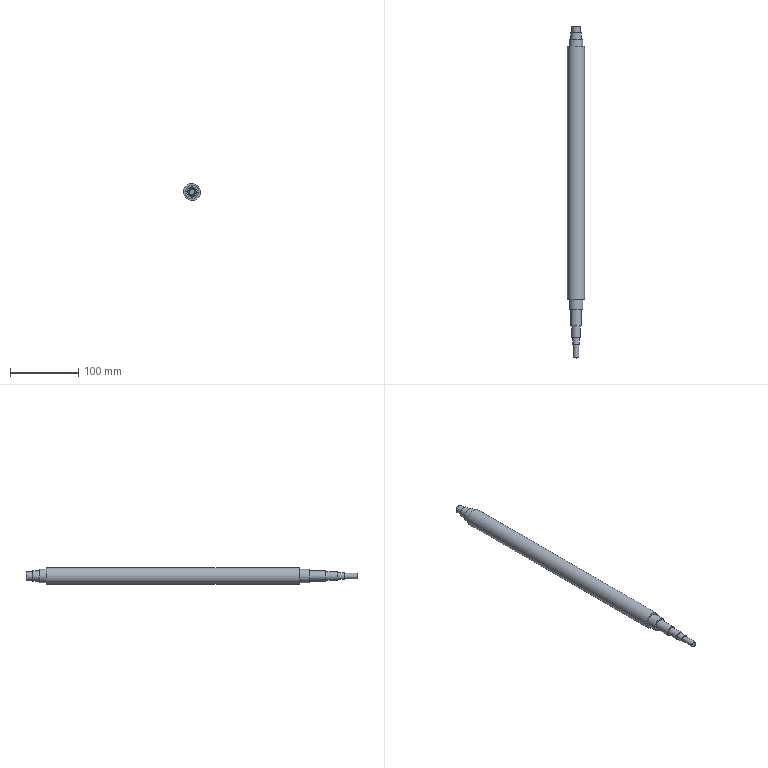Component | NX | Y_LEADSCREW | 1 solid | 19 faces | box 25 x 486 x 25 mm | volume 200330 mm3 | plane 10 | cylinder 9 | commonest cylinder face diameters 12 x2 15 x2 20 x2 8 x1 10 x1 25 x1
STEP:
#1=CARTESIAN_POINT('',(0.,0.,0.));
#2=DIRECTION('',(0.,0.,1.));
#3=DIRECTION('',(1.,0.,0.));
#4=AXIS2_PLACEMENT_3D('',#1,#2,#3);
#5=CARTESIAN_POINT('',(626.907,146.698,-1470.977));
#6=VERTEX_POINT('',#5);
#7=CARTESIAN_POINT('',(630.189,146.698,-1476.));
#8=DIRECTION('',(0.,-1.,0.));
#9=DIRECTION('',(-0.5469,0.,0.8372));
#10=AXIS2_PLACEMENT_3D('',#7,#8,#9);
#11=CIRCLE('',#10,6.);
#12=CARTESIAN_POINT('',(630.189,146.698,-1476.));
#13=DIRECTION('',(0.,-1.,0.));
#14=DIRECTION('',(-0.5469,0.,0.8372));
#15=AXIS2_PLACEMENT_3D('',#12,#13,#14);
#16=PLANE('',#15);
#17=CARTESIAN_POINT('',(0.,0.));
#18=DIRECTION('',(1.,0.));
#19=AXIS2_PLACEMENT_2D('',#17,#18);
#20=CIRCLE('',#19,6.);
#21=(GEOMETRIC_REPRESENTATION_CONTEXT(2)PARAMETRIC_REPRESENTATION_CONTEXT()REPRESENTATION_CONTEXT('',''));
#22=DEFINITIONAL_REPRESENTATION('',(#20),#21);
#23=PCURVE('',#16,#22);
#24=CARTESIAN_POINT('',(630.189,-68.302,-1476.));
#25=DIRECTION('',(0.,-1.,0.));
#26=DIRECTION('',(-0.5469,0.,0.8372));
#27=AXIS2_PLACEMENT_3D('',#24,#25,#26);
#28=CYLINDRICAL_SURFACE('',#27,6.);
#29=CARTESIAN_POINT('',(0.,-215.));
#30=DIRECTION('',(1.,0.));
#31=VECTOR('',#30,1.);
#32=LINE('',#29,#31);
#33=(GEOMETRIC_REPRESENTATION_CONTEXT(2)PARAMETRIC_REPRESENTATION_CONTEXT()REPRESENTATION_CONTEXT('',''));
#34=DEFINITIONAL_REPRESENTATION('',(#32),#33);
#35=PCURVE('',#28,#34);
#36=SURFACE_CURVE('',#11,(#23,#35),.PCURVE_S1.);
#37=EDGE_CURVE('',#6,#6,#36,.T.);
#38=ORIENTED_EDGE('',*,*,#37,.F.);
#39=EDGE_LOOP('',(#38));
#40=FACE_BOUND('',#39,.T.);
#41=ADVANCED_FACE('',(#40),#16,.F.);
#42=CARTESIAN_POINT('',(628.001,-339.302,-1472.651));
#43=VERTEX_POINT('',#42);
#44=CARTESIAN_POINT('',(630.189,-339.302,-1476.));
#45=DIRECTION('',(0.,-1.,0.));
#46=DIRECTION('',(-0.5469,0.,0.8372));
#47=AXIS2_PLACEMENT_3D('',#44,#45,#46);
#48=CIRCLE('',#47,4.);
#49=CARTESIAN_POINT('',(630.189,-339.302,-1476.));
#50=DIRECTION('',(0.,-1.,0.));
#51=DIRECTION('',(-0.5469,0.,0.8372));
#52=AXIS2_PLACEMENT_3D('',#49,#50,#51);
#53=PLANE('',#52);
#54=CARTESIAN_POINT('',(0.,0.));
#55=DIRECTION('',(1.,-0.));
#56=AXIS2_PLACEMENT_2D('',#54,#55);
#57=CIRCLE('',#56,4.);
#58=(GEOMETRIC_REPRESENTATION_CONTEXT(2)PARAMETRIC_REPRESENTATION_CONTEXT()REPRESENTATION_CONTEXT('',''));
#59=DEFINITIONAL_REPRESENTATION('',(#57),#58);
#60=PCURVE('',#53,#59);
#61=CARTESIAN_POINT('',(630.189,-68.302,-1476.));
#62=DIRECTION('',(0.,-1.,0.));
#63=DIRECTION('',(-0.5469,0.,0.8372));
#64=AXIS2_PLACEMENT_3D('',#61,#62,#63);
#65=CYLINDRICAL_SURFACE('',#64,4.);
#66=CARTESIAN_POINT('',(0.,271.));
#67=DIRECTION('',(1.,0.));
#68=VECTOR('',#67,1.);
#69=LINE('',#66,#68);
#70=(GEOMETRIC_REPRESENTATION_CONTEXT(2)PARAMETRIC_REPRESENTATION_CONTEXT()REPRESENTATION_CONTEXT('',''));
#71=DEFINITIONAL_REPRESENTATION('',(#69),#70);
#72=PCURVE('',#65,#71);
#73=SURFACE_CURVE('',#48,(#60,#72),.PCURVE_S1.);
#74=EDGE_CURVE('',#43,#43,#73,.T.);
#75=ORIENTED_EDGE('',*,*,#74,.T.);
#76=EDGE_LOOP('',(#75));
#77=FACE_BOUND('',#76,.T.);
#78=ADVANCED_FACE('',(#77),#53,.T.);
#79=ORIENTED_EDGE('',*,*,#74,.F.);
#80=CARTESIAN_POINT('',(628.001,-319.302,-1472.651));
#81=VERTEX_POINT('',#80);
#82=CARTESIAN_POINT('',(628.001,-319.302,-1472.651));
#83=CARTESIAN_POINT('',(628.001,-339.302,-1472.651));
#84=B_SPLINE_CURVE_WITH_KNOTS('',1,(#82,#83),.UNSPECIFIED.,.F.,.F.,(2,2),(251.,271.),.PIECEWISE_BEZIER_KNOTS.);
#85=CARTESIAN_POINT('',(0.,0.));
#86=DIRECTION('',(0.,1.));
#87=VECTOR('',#86,1.);
#88=LINE('',#85,#87);
#89=(GEOMETRIC_REPRESENTATION_CONTEXT(2)PARAMETRIC_REPRESENTATION_CONTEXT()REPRESENTATION_CONTEXT('',''));
#90=DEFINITIONAL_REPRESENTATION('',(#88),#89);
#91=PCURVE('',#65,#90);
#92=CARTESIAN_POINT('',(6.283,0.));
#93=DIRECTION('',(0.,1.));
#94=VECTOR('',#93,1.);
#95=LINE('',#92,#94);
#96=(GEOMETRIC_REPRESENTATION_CONTEXT(2)PARAMETRIC_REPRESENTATION_CONTEXT()REPRESENTATION_CONTEXT('',''));
#97=DEFINITIONAL_REPRESENTATION('',(#95),#96);
#98=PCURVE('',#65,#97);
#99=SEAM_CURVE('',#84,(#91,#98),.PCURVE_S1.);
#100=EDGE_CURVE('',#81,#43,#99,.T.);
#101=ORIENTED_EDGE('',*,*,#100,.F.);
#102=CARTESIAN_POINT('',(630.189,-319.302,-1476.));
#103=DIRECTION('',(0.,-1.,0.));
#104=DIRECTION('',(-0.5469,0.,0.8372));
#105=AXIS2_PLACEMENT_3D('',#102,#103,#104);
#106=CIRCLE('',#105,4.);
#107=CARTESIAN_POINT('',(0.,251.));
#108=DIRECTION('',(1.,0.));
#109=VECTOR('',#108,1.);
#110=LINE('',#107,#109);
#111=(GEOMETRIC_REPRESENTATION_CONTEXT(2)PARAMETRIC_REPRESENTATION_CONTEXT()REPRESENTATION_CONTEXT('',''));
#112=DEFINITIONAL_REPRESENTATION('',(#110),#111);
#113=PCURVE('',#65,#112);
#114=CARTESIAN_POINT('',(632.924,-319.302,-1480.186));
#115=DIRECTION('',(0.,1.,0.));
#116=DIRECTION('',(0.5469,0.,-0.8372));
#117=AXIS2_PLACEMENT_3D('',#114,#115,#116);
#118=PLANE('',#117);
#119=CARTESIAN_POINT('',(-9.,-0.));
#120=CARTESIAN_POINT('',(-9.,6.928));
#121=CARTESIAN_POINT('',(-3.,3.464));
#122=CARTESIAN_POINT('',(3.,-0.));
#123=CARTESIAN_POINT('',(-3.,-3.464));
#124=CARTESIAN_POINT('',(-9.,-6.928));
#125=CARTESIAN_POINT('',(-9.,-0.));
#126=(BOUNDED_CURVE()B_SPLINE_CURVE(2,(#119,#120,#121,#122,#123,#124,#125),.UNSPECIFIED.,.T.,.F.)B_SPLINE_CURVE_WITH_KNOTS((1,2,2,2,2,1),(-2.094,0.,2.094,4.189,6.283,8.378),.UNSPECIFIED.)CURVE()GEOMETRIC_REPRESENTATION_ITEM()RATIONAL_B_SPLINE_CURVE((1.,0.5,1.,0.5,1.,0.5,1.))REPRESENTATION_ITEM(''));
#127=(GEOMETRIC_REPRESENTATION_CONTEXT(2)PARAMETRIC_REPRESENTATION_CONTEXT()REPRESENTATION_CONTEXT('',''));
#128=DEFINITIONAL_REPRESENTATION('',(#126),#127);
#129=PCURVE('',#118,#128);
#130=SURFACE_CURVE('',#106,(#113,#129),.PCURVE_S1.);
#131=EDGE_CURVE('',#81,#81,#130,.T.);
#132=ORIENTED_EDGE('',*,*,#131,.T.);
#133=ORIENTED_EDGE('',*,*,#100,.T.);
#134=EDGE_LOOP('',(#79,#101,#132,#133));
#135=FACE_BOUND('',#134,.T.);
#136=ADVANCED_FACE('',(#135),#65,.T.);
#137=ORIENTED_EDGE('',*,*,#131,.F.);
#138=EDGE_LOOP('',(#137));
#139=FACE_BOUND('',#138,.T.);
#140=CARTESIAN_POINT('',(627.454,-319.302,-1471.814));
#141=VERTEX_POINT('',#140);
#142=CARTESIAN_POINT('',(630.189,-319.302,-1476.));
#143=DIRECTION('',(0.,-1.,0.));
#144=DIRECTION('',(-0.5469,0.,0.8372));
#145=AXIS2_PLACEMENT_3D('',#142,#143,#144);
#146=CIRCLE('',#145,5.);
#147=CARTESIAN_POINT('',(-10.,-0.));
#148=CARTESIAN_POINT('',(-10.,8.66));
#149=CARTESIAN_POINT('',(-2.5,4.33));
#150=CARTESIAN_POINT('',(5.,-0.));
#151=CARTESIAN_POINT('',(-2.5,-4.33));
#152=CARTESIAN_POINT('',(-10.,-8.66));
#153=CARTESIAN_POINT('',(-10.,-0.));
#154=(BOUNDED_CURVE()B_SPLINE_CURVE(2,(#147,#148,#149,#150,#151,#152,#153),.UNSPECIFIED.,.T.,.F.)B_SPLINE_CURVE_WITH_KNOTS((1,2,2,2,2,1),(-2.094,0.,2.094,4.189,6.283,8.378),.UNSPECIFIED.)CURVE()GEOMETRIC_REPRESENTATION_ITEM()RATIONAL_B_SPLINE_CURVE((1.,0.5,1.,0.5,1.,0.5,1.))REPRESENTATION_ITEM(''));
#155=(GEOMETRIC_REPRESENTATION_CONTEXT(2)PARAMETRIC_REPRESENTATION_CONTEXT()REPRESENTATION_CONTEXT('',''));
#156=DEFINITIONAL_REPRESENTATION('',(#154),#155);
#157=PCURVE('',#118,#156);
#158=CARTESIAN_POINT('',(630.189,-68.302,-1476.));
#159=DIRECTION('',(0.,-1.,0.));
#160=DIRECTION('',(-0.5469,0.,0.8372));
#161=AXIS2_PLACEMENT_3D('',#158,#159,#160);
#162=CYLINDRICAL_SURFACE('',#161,5.);
#163=CARTESIAN_POINT('',(0.,251.));
#164=DIRECTION('',(1.,0.));
#165=VECTOR('',#164,1.);
#166=LINE('',#163,#165);
#167=(GEOMETRIC_REPRESENTATION_CONTEXT(2)PARAMETRIC_REPRESENTATION_CONTEXT()REPRESENTATION_CONTEXT('',''));
#168=DEFINITIONAL_REPRESENTATION('',(#166),#167);
#169=PCURVE('',#162,#168);
#170=SURFACE_CURVE('',#146,(#157,#169),.PCURVE_S1.);
#171=EDGE_CURVE('',#141,#141,#170,.T.);
#172=ORIENTED_EDGE('',*,*,#171,.T.);
#173=EDGE_LOOP('',(#172));
#174=FACE_BOUND('',#173,.T.);
#175=ADVANCED_FACE('',(#139,#174),#118,.F.);
#176=ORIENTED_EDGE('',*,*,#171,.F.);
#177=CARTESIAN_POINT('',(627.454,-309.302,-1471.814));
#178=VERTEX_POINT('',#177);
#179=CARTESIAN_POINT('',(627.454,-309.302,-1471.814));
#180=CARTESIAN_POINT('',(627.454,-319.302,-1471.814));
#181=B_SPLINE_CURVE_WITH_KNOTS('',1,(#179,#180),.UNSPECIFIED.,.F.,.F.,(2,2),(241.,251.),.PIECEWISE_BEZIER_KNOTS.);
#182=CARTESIAN_POINT('',(0.,0.));
#183=DIRECTION('',(0.,1.));
#184=VECTOR('',#183,1.);
#185=LINE('',#182,#184);
#186=(GEOMETRIC_REPRESENTATION_CONTEXT(2)PARAMETRIC_REPRESENTATION_CONTEXT()REPRESENTATION_CONTEXT('',''));
#187=DEFINITIONAL_REPRESENTATION('',(#185),#186);
#188=PCURVE('',#162,#187);
#189=CARTESIAN_POINT('',(6.283,0.));
#190=DIRECTION('',(0.,1.));
#191=VECTOR('',#190,1.);
#192=LINE('',#189,#191);
#193=(GEOMETRIC_REPRESENTATION_CONTEXT(2)PARAMETRIC_REPRESENTATION_CONTEXT()REPRESENTATION_CONTEXT('',''));
#194=DEFINITIONAL_REPRESENTATION('',(#192),#193);
#195=PCURVE('',#162,#194);
#196=SEAM_CURVE('',#181,(#188,#195),.PCURVE_S1.);
#197=EDGE_CURVE('',#178,#141,#196,.T.);
#198=ORIENTED_EDGE('',*,*,#197,.F.);
#199=CARTESIAN_POINT('',(630.189,-309.302,-1476.));
#200=DIRECTION('',(0.,-1.,0.));
#201=DIRECTION('',(-0.5469,0.,0.8372));
#202=AXIS2_PLACEMENT_3D('',#199,#200,#201);
#203=CIRCLE('',#202,5.);
#204=CARTESIAN_POINT('',(0.,241.));
#205=DIRECTION('',(1.,0.));
#206=VECTOR('',#205,1.);
#207=LINE('',#204,#206);
#208=(GEOMETRIC_REPRESENTATION_CONTEXT(2)PARAMETRIC_REPRESENTATION_CONTEXT()REPRESENTATION_CONTEXT('',''));
#209=DEFINITIONAL_REPRESENTATION('',(#207),#208);
#210=PCURVE('',#162,#209);
#211=CARTESIAN_POINT('',(633.471,-309.302,-1481.023));
#212=DIRECTION('',(0.,1.,0.));
#213=DIRECTION('',(0.5469,0.,-0.8372));
#214=AXIS2_PLACEMENT_3D('',#211,#212,#213);
#215=PLANE('',#214);
#216=CARTESIAN_POINT('',(-11.,-0.));
#217=CARTESIAN_POINT('',(-11.,8.66));
#218=CARTESIAN_POINT('',(-3.5,4.33));
#219=CARTESIAN_POINT('',(4.,-0.));
#220=CARTESIAN_POINT('',(-3.5,-4.33));
#221=CARTESIAN_POINT('',(-11.,-8.66));
#222=CARTESIAN_POINT('',(-11.,-0.));
#223=(BOUNDED_CURVE()B_SPLINE_CURVE(2,(#216,#217,#218,#219,#220,#221,#222),.UNSPECIFIED.,.T.,.F.)B_SPLINE_CURVE_WITH_KNOTS((1,2,2,2,2,1),(-2.094,0.,2.094,4.189,6.283,8.378),.UNSPECIFIED.)CURVE()GEOMETRIC_REPRESENTATION_ITEM()RATIONAL_B_SPLINE_CURVE((1.,0.5,1.,0.5,1.,0.5,1.))REPRESENTATION_ITEM(''));
#224=(GEOMETRIC_REPRESENTATION_CONTEXT(2)PARAMETRIC_REPRESENTATION_CONTEXT()REPRESENTATION_CONTEXT('',''));
#225=DEFINITIONAL_REPRESENTATION('',(#223),#224);
#226=PCURVE('',#215,#225);
#227=SURFACE_CURVE('',#203,(#210,#226),.PCURVE_S1.);
#228=EDGE_CURVE('',#178,#178,#227,.T.);
#229=ORIENTED_EDGE('',*,*,#228,.T.);
#230=ORIENTED_EDGE('',*,*,#197,.T.);
#231=EDGE_LOOP('',(#176,#198,#229,#230));
#232=FACE_BOUND('',#231,.T.);
#233=ADVANCED_FACE('',(#232),#162,.T.);
#234=ORIENTED_EDGE('',*,*,#228,.F.);
#235=EDGE_LOOP('',(#234));
#236=FACE_BOUND('',#235,.T.);
#237=CARTESIAN_POINT('',(626.907,-309.302,-1470.977));
#238=VERTEX_POINT('',#237);
#239=CARTESIAN_POINT('',(630.189,-309.302,-1476.));
#240=DIRECTION('',(0.,-1.,0.));
#241=DIRECTION('',(-0.5469,0.,0.8372));
#242=AXIS2_PLACEMENT_3D('',#239,#240,#241);
#243=CIRCLE('',#242,6.);
#244=CARTESIAN_POINT('',(-12.,-0.));
#245=CARTESIAN_POINT('',(-12.,10.392));
#246=CARTESIAN_POINT('',(-3.,5.196));
#247=CARTESIAN_POINT('',(6.,-0.));
#248=CARTESIAN_POINT('',(-3.,-5.196));
#249=CARTESIAN_POINT('',(-12.,-10.392));
#250=CARTESIAN_POINT('',(-12.,-0.));
#251=(BOUNDED_CURVE()B_SPLINE_CURVE(2,(#244,#245,#246,#247,#248,#249,#250),.UNSPECIFIED.,.T.,.F.)B_SPLINE_CURVE_WITH_KNOTS((1,2,2,2,2,1),(-2.094,0.,2.094,4.189,6.283,8.378),.UNSPECIFIED.)CURVE()GEOMETRIC_REPRESENTATION_ITEM()RATIONAL_B_SPLINE_CURVE((1.,0.5,1.,0.5,1.,0.5,1.))REPRESENTATION_ITEM(''));
#252=(GEOMETRIC_REPRESENTATION_CONTEXT(2)PARAMETRIC_REPRESENTATION_CONTEXT()REPRESENTATION_CONTEXT('',''));
#253=DEFINITIONAL_REPRESENTATION('',(#251),#252);
#254=PCURVE('',#215,#253);
#255=CARTESIAN_POINT('',(630.189,-68.302,-1476.));
#256=DIRECTION('',(0.,-1.,0.));
#257=DIRECTION('',(-0.5469,0.,0.8372));
#258=AXIS2_PLACEMENT_3D('',#255,#256,#257);
#259=CYLINDRICAL_SURFACE('',#258,6.);
#260=CARTESIAN_POINT('',(0.,241.));
#261=DIRECTION('',(1.,0.));
#262=VECTOR('',#261,1.);
#263=LINE('',#260,#262);
#264=(GEOMETRIC_REPRESENTATION_CONTEXT(2)PARAMETRIC_REPRESENTATION_CONTEXT()REPRESENTATION_CONTEXT('',''));
#265=DEFINITIONAL_REPRESENTATION('',(#263),#264);
#266=PCURVE('',#259,#265);
#267=SURFACE_CURVE('',#243,(#254,#266),.PCURVE_S1.);
#268=EDGE_CURVE('',#238,#238,#267,.T.);
#269=ORIENTED_EDGE('',*,*,#268,.T.);
#270=EDGE_LOOP('',(#269));
#271=FACE_BOUND('',#270,.T.);
#272=ADVANCED_FACE('',(#236,#271),#215,.F.);
#273=ORIENTED_EDGE('',*,*,#268,.F.);
#274=CARTESIAN_POINT('',(626.907,-292.302,-1470.977));
#275=VERTEX_POINT('',#274);
#276=CARTESIAN_POINT('',(626.907,-292.302,-1470.977));
#277=CARTESIAN_POINT('',(626.907,-309.302,-1470.977));
#278=B_SPLINE_CURVE_WITH_KNOTS('',1,(#276,#277),.UNSPECIFIED.,.F.,.F.,(2,2),(224.,241.),.PIECEWISE_BEZIER_KNOTS.);
#279=CARTESIAN_POINT('',(0.,0.));
#280=DIRECTION('',(0.,1.));
#281=VECTOR('',#280,1.);
#282=LINE('',#279,#281);
#283=(GEOMETRIC_REPRESENTATION_CONTEXT(2)PARAMETRIC_REPRESENTATION_CONTEXT()REPRESENTATION_CONTEXT('',''));
#284=DEFINITIONAL_REPRESENTATION('',(#282),#283);
#285=PCURVE('',#259,#284);
#286=CARTESIAN_POINT('',(6.283,0.));
#287=DIRECTION('',(0.,1.));
#288=VECTOR('',#287,1.);
#289=LINE('',#286,#288);
#290=(GEOMETRIC_REPRESENTATION_CONTEXT(2)PARAMETRIC_REPRESENTATION_CONTEXT()REPRESENTATION_CONTEXT('',''));
#291=DEFINITIONAL_REPRESENTATION('',(#289),#290);
#292=PCURVE('',#259,#291);
#293=SEAM_CURVE('',#278,(#285,#292),.PCURVE_S1.);
#294=EDGE_CURVE('',#275,#238,#293,.T.);
#295=ORIENTED_EDGE('',*,*,#294,.F.);
#296=CARTESIAN_POINT('',(630.189,-292.302,-1476.));
#297=DIRECTION('',(0.,-1.,0.));
#298=DIRECTION('',(-0.5469,0.,0.8372));
#299=AXIS2_PLACEMENT_3D('',#296,#297,#298);
#300=CIRCLE('',#299,6.);
#301=CARTESIAN_POINT('',(0.,224.));
#302=DIRECTION('',(1.,0.));
#303=VECTOR('',#302,1.);
#304=LINE('',#301,#303);
#305=(GEOMETRIC_REPRESENTATION_CONTEXT(2)PARAMETRIC_REPRESENTATION_CONTEXT()REPRESENTATION_CONTEXT('',''));
#306=DEFINITIONAL_REPRESENTATION('',(#304),#305);
#307=PCURVE('',#259,#306);
#308=CARTESIAN_POINT('',(634.291,-292.302,-1482.279));
#309=DIRECTION('',(0.,1.,0.));
#310=DIRECTION('',(0.5469,0.,-0.8372));
#311=AXIS2_PLACEMENT_3D('',#308,#309,#310);
#312=PLANE('',#311);
#313=CARTESIAN_POINT('',(-13.5,0.));
#314=CARTESIAN_POINT('',(-13.5,10.392));
#315=CARTESIAN_POINT('',(-4.5,5.196));
#316=CARTESIAN_POINT('',(4.5,0.));
#317=CARTESIAN_POINT('',(-4.5,-5.196));
#318=CARTESIAN_POINT('',(-13.5,-10.392));
#319=CARTESIAN_POINT('',(-13.5,0.));
#320=(BOUNDED_CURVE()B_SPLINE_CURVE(2,(#313,#314,#315,#316,#317,#318,#319),.UNSPECIFIED.,.T.,.F.)B_SPLINE_CURVE_WITH_KNOTS((1,2,2,2,2,1),(-2.094,0.,2.094,4.189,6.283,8.378),.UNSPECIFIED.)CURVE()GEOMETRIC_REPRESENTATION_ITEM()RATIONAL_B_SPLINE_CURVE((1.,0.5,1.,0.5,1.,0.5,1.))REPRESENTATION_ITEM(''));
#321=(GEOMETRIC_REPRESENTATION_CONTEXT(2)PARAMETRIC_REPRESENTATION_CONTEXT()REPRESENTATION_CONTEXT('',''));
#322=DEFINITIONAL_REPRESENTATION('',(#320),#321);
#323=PCURVE('',#312,#322);
#324=SURFACE_CURVE('',#300,(#307,#323),.PCURVE_S1.);
#325=EDGE_CURVE('',#275,#275,#324,.T.);
#326=ORIENTED_EDGE('',*,*,#325,.T.);
#327=ORIENTED_EDGE('',*,*,#294,.T.);
#328=EDGE_LOOP('',(#273,#295,#326,#327));
#329=FACE_BOUND('',#328,.T.);
#330=ADVANCED_FACE('',(#329),#259,.T.);
#331=ORIENTED_EDGE('',*,*,#325,.F.);
#332=EDGE_LOOP('',(#331));
#333=FACE_BOUND('',#332,.T.);
#334=CARTESIAN_POINT('',(626.087,-292.302,-1469.721));
#335=VERTEX_POINT('',#334);
#336=CARTESIAN_POINT('',(630.189,-292.302,-1476.));
#337=DIRECTION('',(0.,-1.,0.));
#338=DIRECTION('',(-0.5469,0.,0.8372));
#339=AXIS2_PLACEMENT_3D('',#336,#337,#338);
#340=CIRCLE('',#339,7.5);
#341=CARTESIAN_POINT('',(-15.,0.));
#342=CARTESIAN_POINT('',(-15.,12.99));
#343=CARTESIAN_POINT('',(-3.75,6.495));
#344=CARTESIAN_POINT('',(7.5,0.));
#345=CARTESIAN_POINT('',(-3.75,-6.495));
#346=CARTESIAN_POINT('',(-15.,-12.99));
#347=CARTESIAN_POINT('',(-15.,0.));
#348=(BOUNDED_CURVE()B_SPLINE_CURVE(2,(#341,#342,#343,#344,#345,#346,#347),.UNSPECIFIED.,.T.,.F.)B_SPLINE_CURVE_WITH_KNOTS((1,2,2,2,2,1),(-2.094,0.,2.094,4.189,6.283,8.378),.UNSPECIFIED.)CURVE()GEOMETRIC_REPRESENTATION_ITEM()RATIONAL_B_SPLINE_CURVE((1.,0.5,1.,0.5,1.,0.5,1.))REPRESENTATION_ITEM(''));
#349=(GEOMETRIC_REPRESENTATION_CONTEXT(2)PARAMETRIC_REPRESENTATION_CONTEXT()REPRESENTATION_CONTEXT('',''));
#350=DEFINITIONAL_REPRESENTATION('',(#348),#349);
#351=PCURVE('',#312,#350);
#352=CARTESIAN_POINT('',(630.189,-68.302,-1476.));
#353=DIRECTION('',(0.,-1.,0.));
#354=DIRECTION('',(-0.5469,0.,0.8372));
#355=AXIS2_PLACEMENT_3D('',#352,#353,#354);
#356=CYLINDRICAL_SURFACE('',#355,7.5);
#357=CARTESIAN_POINT('',(0.,224.));
#358=DIRECTION('',(1.,0.));
#359=VECTOR('',#358,1.);
#360=LINE('',#357,#359);
#361=(GEOMETRIC_REPRESENTATION_CONTEXT(2)PARAMETRIC_REPRESENTATION_CONTEXT()REPRESENTATION_CONTEXT('',''));
#362=DEFINITIONAL_REPRESENTATION('',(#360),#361);
#363=PCURVE('',#356,#362);
#364=SURFACE_CURVE('',#340,(#351,#363),.PCURVE_S1.);
#365=EDGE_CURVE('',#335,#335,#364,.T.);
#366=ORIENTED_EDGE('',*,*,#365,.T.);
#367=EDGE_LOOP('',(#366));
#368=FACE_BOUND('',#367,.T.);
#369=ADVANCED_FACE('',(#333,#368),#312,.F.);
#370=ORIENTED_EDGE('',*,*,#365,.F.);
#371=CARTESIAN_POINT('',(626.087,-268.302,-1469.721));
#372=VERTEX_POINT('',#371);
#373=CARTESIAN_POINT('',(626.087,-268.302,-1469.721));
#374=CARTESIAN_POINT('',(626.087,-292.302,-1469.721));
#375=B_SPLINE_CURVE_WITH_KNOTS('',1,(#373,#374),.UNSPECIFIED.,.F.,.F.,(2,2),(200.,224.),.PIECEWISE_BEZIER_KNOTS.);
#376=CARTESIAN_POINT('',(0.,0.));
#377=DIRECTION('',(0.,1.));
#378=VECTOR('',#377,1.);
#379=LINE('',#376,#378);
#380=(GEOMETRIC_REPRESENTATION_CONTEXT(2)PARAMETRIC_REPRESENTATION_CONTEXT()REPRESENTATION_CONTEXT('',''));
#381=DEFINITIONAL_REPRESENTATION('',(#379),#380);
#382=PCURVE('',#356,#381);
#383=CARTESIAN_POINT('',(6.283,0.));
#384=DIRECTION('',(0.,1.));
#385=VECTOR('',#384,1.);
#386=LINE('',#383,#385);
#387=(GEOMETRIC_REPRESENTATION_CONTEXT(2)PARAMETRIC_REPRESENTATION_CONTEXT()REPRESENTATION_CONTEXT('',''));
#388=DEFINITIONAL_REPRESENTATION('',(#386),#387);
#389=PCURVE('',#356,#388);
#390=SEAM_CURVE('',#375,(#382,#389),.PCURVE_S1.);
#391=EDGE_CURVE('',#372,#335,#390,.T.);
#392=ORIENTED_EDGE('',*,*,#391,.F.);
#393=CARTESIAN_POINT('',(630.189,-268.302,-1476.));
#394=DIRECTION('',(0.,-1.,0.));
#395=DIRECTION('',(-0.5469,0.,0.8372));
#396=AXIS2_PLACEMENT_3D('',#393,#394,#395);
#397=CIRCLE('',#396,7.5);
#398=CARTESIAN_POINT('',(0.,200.));
#399=DIRECTION('',(1.,0.));
#400=VECTOR('',#399,1.);
#401=LINE('',#398,#400);
#402=(GEOMETRIC_REPRESENTATION_CONTEXT(2)PARAMETRIC_REPRESENTATION_CONTEXT()REPRESENTATION_CONTEXT('',''));
#403=DEFINITIONAL_REPRESENTATION('',(#401),#402);
#404=PCURVE('',#356,#403);
#405=CARTESIAN_POINT('',(635.658,-268.302,-1484.372));
#406=DIRECTION('',(0.,1.,0.));
#407=DIRECTION('',(0.5469,0.,-0.8372));
#408=AXIS2_PLACEMENT_3D('',#405,#406,#407);
#409=PLANE('',#408);
#410=CARTESIAN_POINT('',(-17.5,0.));
#411=CARTESIAN_POINT('',(-17.5,12.99));
#412=CARTESIAN_POINT('',(-6.25,6.495));
#413=CARTESIAN_POINT('',(5.,0.));
#414=CARTESIAN_POINT('',(-6.25,-6.495));
#415=CARTESIAN_POINT('',(-17.5,-12.99));
#416=CARTESIAN_POINT('',(-17.5,0.));
#417=(BOUNDED_CURVE()B_SPLINE_CURVE(2,(#410,#411,#412,#413,#414,#415,#416),.UNSPECIFIED.,.T.,.F.)B_SPLINE_CURVE_WITH_KNOTS((1,2,2,2,2,1),(-2.094,0.,2.094,4.189,6.283,8.378),.UNSPECIFIED.)CURVE()GEOMETRIC_REPRESENTATION_ITEM()RATIONAL_B_SPLINE_CURVE((1.,0.5,1.,0.5,1.,0.5,1.))REPRESENTATION_ITEM(''));
#418=(GEOMETRIC_REPRESENTATION_CONTEXT(2)PARAMETRIC_REPRESENTATION_CONTEXT()REPRESENTATION_CONTEXT('',''));
#419=DEFINITIONAL_REPRESENTATION('',(#417),#418);
#420=PCURVE('',#409,#419);
#421=SURFACE_CURVE('',#397,(#404,#420),.PCURVE_S1.);
#422=EDGE_CURVE('',#372,#372,#421,.T.);
#423=ORIENTED_EDGE('',*,*,#422,.T.);
#424=ORIENTED_EDGE('',*,*,#391,.T.);
#425=EDGE_LOOP('',(#370,#392,#423,#424));
#426=FACE_BOUND('',#425,.T.);
#427=ADVANCED_FACE('',(#426),#356,.T.);
#428=ORIENTED_EDGE('',*,*,#422,.F.);
#429=EDGE_LOOP('',(#428));
#430=FACE_BOUND('',#429,.T.);
#431=CARTESIAN_POINT('',(624.72,-268.302,-1467.628));
#432=VERTEX_POINT('',#431);
#433=CARTESIAN_POINT('',(630.189,-268.302,-1476.));
#434=DIRECTION('',(0.,-1.,0.));
#435=DIRECTION('',(-0.5469,0.,0.8372));
#436=AXIS2_PLACEMENT_3D('',#433,#434,#435);
#437=CIRCLE('',#436,10.);
#438=CARTESIAN_POINT('',(-20.,0.));
#439=CARTESIAN_POINT('',(-20.,17.321));
#440=CARTESIAN_POINT('',(-5.,8.66));
#441=CARTESIAN_POINT('',(10.,0.));
#442=CARTESIAN_POINT('',(-5.,-8.66));
#443=CARTESIAN_POINT('',(-20.,-17.321));
#444=CARTESIAN_POINT('',(-20.,0.));
#445=(BOUNDED_CURVE()B_SPLINE_CURVE(2,(#438,#439,#440,#441,#442,#443,#444),.UNSPECIFIED.,.T.,.F.)B_SPLINE_CURVE_WITH_KNOTS((1,2,2,2,2,1),(-2.094,0.,2.094,4.189,6.283,8.378),.UNSPECIFIED.)CURVE()GEOMETRIC_REPRESENTATION_ITEM()RATIONAL_B_SPLINE_CURVE((1.,0.5,1.,0.5,1.,0.5,1.))REPRESENTATION_ITEM(''));
#446=(GEOMETRIC_REPRESENTATION_CONTEXT(2)PARAMETRIC_REPRESENTATION_CONTEXT()REPRESENTATION_CONTEXT('',''));
#447=DEFINITIONAL_REPRESENTATION('',(#445),#446);
#448=PCURVE('',#409,#447);
#449=CARTESIAN_POINT('',(630.189,-68.302,-1476.));
#450=DIRECTION('',(0.,-1.,0.));
#451=DIRECTION('',(-0.5469,0.,0.8372));
#452=AXIS2_PLACEMENT_3D('',#449,#450,#451);
#453=CYLINDRICAL_SURFACE('',#452,10.);
#454=CARTESIAN_POINT('',(0.,200.));
#455=DIRECTION('',(1.,0.));
#456=VECTOR('',#455,1.);
#457=LINE('',#454,#456);
#458=(GEOMETRIC_REPRESENTATION_CONTEXT(2)PARAMETRIC_REPRESENTATION_CONTEXT()REPRESENTATION_CONTEXT('',''));
#459=DEFINITIONAL_REPRESENTATION('',(#457),#458);
#460=PCURVE('',#453,#459);
#461=SURFACE_CURVE('',#437,(#448,#460),.PCURVE_S1.);
#462=EDGE_CURVE('',#432,#432,#461,.T.);
#463=ORIENTED_EDGE('',*,*,#462,.T.);
#464=EDGE_LOOP('',(#463));
#465=FACE_BOUND('',#464,.T.);
#466=ADVANCED_FACE('',(#430,#465),#409,.F.);
#467=ORIENTED_EDGE('',*,*,#462,.F.);
#468=CARTESIAN_POINT('',(624.72,-253.302,-1467.628));
#469=VERTEX_POINT('',#468);
#470=CARTESIAN_POINT('',(624.72,-253.302,-1467.628));
#471=CARTESIAN_POINT('',(624.72,-268.302,-1467.628));
#472=B_SPLINE_CURVE_WITH_KNOTS('',1,(#470,#471),.UNSPECIFIED.,.F.,.F.,(2,2),(185.,200.),.PIECEWISE_BEZIER_KNOTS.);
#473=CARTESIAN_POINT('',(0.,0.));
#474=DIRECTION('',(0.,1.));
#475=VECTOR('',#474,1.);
#476=LINE('',#473,#475);
#477=(GEOMETRIC_REPRESENTATION_CONTEXT(2)PARAMETRIC_REPRESENTATION_CONTEXT()REPRESENTATION_CONTEXT('',''));
#478=DEFINITIONAL_REPRESENTATION('',(#476),#477);
#479=PCURVE('',#453,#478);
#480=CARTESIAN_POINT('',(6.283,0.));
#481=DIRECTION('',(0.,1.));
#482=VECTOR('',#481,1.);
#483=LINE('',#480,#482);
#484=(GEOMETRIC_REPRESENTATION_CONTEXT(2)PARAMETRIC_REPRESENTATION_CONTEXT()REPRESENTATION_CONTEXT('',''));
#485=DEFINITIONAL_REPRESENTATION('',(#483),#484);
#486=PCURVE('',#453,#485);
#487=SEAM_CURVE('',#472,(#479,#486),.PCURVE_S1.);
#488=EDGE_CURVE('',#469,#432,#487,.T.);
#489=ORIENTED_EDGE('',*,*,#488,.F.);
#490=CARTESIAN_POINT('',(630.189,-253.302,-1476.));
#491=DIRECTION('',(0.,-1.,0.));
#492=DIRECTION('',(-0.5469,0.,0.8372));
#493=AXIS2_PLACEMENT_3D('',#490,#491,#492);
#494=CIRCLE('',#493,10.);
#495=CARTESIAN_POINT('',(0.,185.));
#496=DIRECTION('',(1.,0.));
#497=VECTOR('',#496,1.);
#498=LINE('',#495,#497);
#499=(GEOMETRIC_REPRESENTATION_CONTEXT(2)PARAMETRIC_REPRESENTATION_CONTEXT()REPRESENTATION_CONTEXT('',''));
#500=DEFINITIONAL_REPRESENTATION('',(#498),#499);
#501=PCURVE('',#453,#500);
#502=CARTESIAN_POINT('',(637.026,-253.302,-1486.465));
#503=DIRECTION('',(0.,1.,0.));
#504=DIRECTION('',(0.5469,0.,-0.8372));
#505=AXIS2_PLACEMENT_3D('',#502,#503,#504);
#506=PLANE('',#505);
#507=CARTESIAN_POINT('',(-22.5,0.));
#508=CARTESIAN_POINT('',(-22.5,17.321));
#509=CARTESIAN_POINT('',(-7.5,8.66));
#510=CARTESIAN_POINT('',(7.5,0.));
#511=CARTESIAN_POINT('',(-7.5,-8.66));
#512=CARTESIAN_POINT('',(-22.5,-17.321));
#513=CARTESIAN_POINT('',(-22.5,0.));
#514=(BOUNDED_CURVE()B_SPLINE_CURVE(2,(#507,#508,#509,#510,#511,#512,#513),.UNSPECIFIED.,.T.,.F.)B_SPLINE_CURVE_WITH_KNOTS((1,2,2,2,2,1),(-2.094,0.,2.094,4.189,6.283,8.378),.UNSPECIFIED.)CURVE()GEOMETRIC_REPRESENTATION_ITEM()RATIONAL_B_SPLINE_CURVE((1.,0.5,1.,0.5,1.,0.5,1.))REPRESENTATION_ITEM(''));
#515=(GEOMETRIC_REPRESENTATION_CONTEXT(2)PARAMETRIC_REPRESENTATION_CONTEXT()REPRESENTATION_CONTEXT('',''));
#516=DEFINITIONAL_REPRESENTATION('',(#514),#515);
#517=PCURVE('',#506,#516);
#518=SURFACE_CURVE('',#494,(#501,#517),.PCURVE_S1.);
#519=EDGE_CURVE('',#469,#469,#518,.T.);
#520=ORIENTED_EDGE('',*,*,#519,.T.);
#521=ORIENTED_EDGE('',*,*,#488,.T.);
#522=EDGE_LOOP('',(#467,#489,#520,#521));
#523=FACE_BOUND('',#522,.T.);
#524=ADVANCED_FACE('',(#523),#453,.T.);
#525=ORIENTED_EDGE('',*,*,#519,.F.);
#526=EDGE_LOOP('',(#525));
#527=FACE_BOUND('',#526,.T.);
#528=CARTESIAN_POINT('',(623.352,-253.302,-1465.535));
#529=VERTEX_POINT('',#528);
#530=CARTESIAN_POINT('',(630.189,-253.302,-1476.));
#531=DIRECTION('',(0.,-1.,0.));
#532=DIRECTION('',(-0.5469,0.,0.8372));
#533=AXIS2_PLACEMENT_3D('',#530,#531,#532);
#534=CIRCLE('',#533,12.5);
#535=CARTESIAN_POINT('',(-25.,0.));
#536=CARTESIAN_POINT('',(-25.,21.651));
#537=CARTESIAN_POINT('',(-6.25,10.825));
#538=CARTESIAN_POINT('',(12.5,0.));
#539=CARTESIAN_POINT('',(-6.25,-10.825));
#540=CARTESIAN_POINT('',(-25.,-21.651));
#541=CARTESIAN_POINT('',(-25.,0.));
#542=(BOUNDED_CURVE()B_SPLINE_CURVE(2,(#535,#536,#537,#538,#539,#540,#541),.UNSPECIFIED.,.T.,.F.)B_SPLINE_CURVE_WITH_KNOTS((1,2,2,2,2,1),(-2.094,0.,2.094,4.189,6.283,8.378),.UNSPECIFIED.)CURVE()GEOMETRIC_REPRESENTATION_ITEM()RATIONAL_B_SPLINE_CURVE((1.,0.5,1.,0.5,1.,0.5,1.))REPRESENTATION_ITEM(''));
#543=(GEOMETRIC_REPRESENTATION_CONTEXT(2)PARAMETRIC_REPRESENTATION_CONTEXT()REPRESENTATION_CONTEXT('',''));
#544=DEFINITIONAL_REPRESENTATION('',(#542),#543);
#545=PCURVE('',#506,#544);
#546=CARTESIAN_POINT('',(630.189,-68.302,-1476.));
#547=DIRECTION('',(0.,-1.,0.));
#548=DIRECTION('',(-0.5469,0.,0.8372));
#549=AXIS2_PLACEMENT_3D('',#546,#547,#548);
#550=CYLINDRICAL_SURFACE('',#549,12.5);
#551=CARTESIAN_POINT('',(0.,185.));
#552=DIRECTION('',(1.,0.));
#553=VECTOR('',#552,1.);
#554=LINE('',#551,#553);
#555=(GEOMETRIC_REPRESENTATION_CONTEXT(2)PARAMETRIC_REPRESENTATION_CONTEXT()REPRESENTATION_CONTEXT('',''));
#556=DEFINITIONAL_REPRESENTATION('',(#554),#555);
#557=PCURVE('',#550,#556);
#558=SURFACE_CURVE('',#534,(#545,#557),.PCURVE_S1.);
#559=EDGE_CURVE('',#529,#529,#558,.T.);
#560=ORIENTED_EDGE('',*,*,#559,.T.);
#561=EDGE_LOOP('',(#560));
#562=FACE_BOUND('',#561,.T.);
#563=ADVANCED_FACE('',(#527,#562),#506,.F.);
#564=ORIENTED_EDGE('',*,*,#559,.F.);
#565=CARTESIAN_POINT('',(623.352,116.698,-1465.535));
#566=VERTEX_POINT('',#565);
#567=CARTESIAN_POINT('',(623.352,116.698,-1465.535));
#568=CARTESIAN_POINT('',(623.352,-253.302,-1465.535));
#569=B_SPLINE_CURVE_WITH_KNOTS('',1,(#567,#568),.UNSPECIFIED.,.F.,.F.,(2,2),(-185.,185.),.PIECEWISE_BEZIER_KNOTS.);
#570=CARTESIAN_POINT('',(0.,0.));
#571=DIRECTION('',(0.,1.));
#572=VECTOR('',#571,1.);
#573=LINE('',#570,#572);
#574=(GEOMETRIC_REPRESENTATION_CONTEXT(2)PARAMETRIC_REPRESENTATION_CONTEXT()REPRESENTATION_CONTEXT('',''));
#575=DEFINITIONAL_REPRESENTATION('',(#573),#574);
#576=PCURVE('',#550,#575);
#577=CARTESIAN_POINT('',(6.283,0.));
#578=DIRECTION('',(0.,1.));
#579=VECTOR('',#578,1.);
#580=LINE('',#577,#579);
#581=(GEOMETRIC_REPRESENTATION_CONTEXT(2)PARAMETRIC_REPRESENTATION_CONTEXT()REPRESENTATION_CONTEXT('',''));
#582=DEFINITIONAL_REPRESENTATION('',(#580),#581);
#583=PCURVE('',#550,#582);
#584=SEAM_CURVE('',#569,(#576,#583),.PCURVE_S1.);
#585=EDGE_CURVE('',#566,#529,#584,.T.);
#586=ORIENTED_EDGE('',*,*,#585,.F.);
#587=CARTESIAN_POINT('',(630.189,116.698,-1476.));
#588=DIRECTION('',(0.,-1.,0.));
#589=DIRECTION('',(-0.5469,0.,0.8372));
#590=AXIS2_PLACEMENT_3D('',#587,#588,#589);
#591=CIRCLE('',#590,12.5);
#592=CARTESIAN_POINT('',(0.,-185.));
#593=DIRECTION('',(1.,0.));
#594=VECTOR('',#593,1.);
#595=LINE('',#592,#594);
#596=(GEOMETRIC_REPRESENTATION_CONTEXT(2)PARAMETRIC_REPRESENTATION_CONTEXT()REPRESENTATION_CONTEXT('',''));
#597=DEFINITIONAL_REPRESENTATION('',(#595),#596);
#598=PCURVE('',#550,#597);
#599=CARTESIAN_POINT('',(635.658,116.698,-1484.372));
#600=DIRECTION('',(0.,-1.,0.));
#601=DIRECTION('',(-0.5469,0.,0.8372));
#602=AXIS2_PLACEMENT_3D('',#599,#600,#601);
#603=PLANE('',#602);
#604=CARTESIAN_POINT('',(10.,0.));
#605=DIRECTION('',(1.,0.));
#606=AXIS2_PLACEMENT_2D('',#604,#605);
#607=CIRCLE('',#606,12.5);
#608=(GEOMETRIC_REPRESENTATION_CONTEXT(2)PARAMETRIC_REPRESENTATION_CONTEXT()REPRESENTATION_CONTEXT('',''));
#609=DEFINITIONAL_REPRESENTATION('',(#607),#608);
#610=PCURVE('',#603,#609);
#611=SURFACE_CURVE('',#591,(#598,#610),.PCURVE_S1.);
#612=EDGE_CURVE('',#566,#566,#611,.T.);
#613=ORIENTED_EDGE('',*,*,#612,.T.);
#614=ORIENTED_EDGE('',*,*,#585,.T.);
#615=EDGE_LOOP('',(#564,#586,#613,#614));
#616=FACE_BOUND('',#615,.T.);
#617=ADVANCED_FACE('',(#616),#550,.T.);
#618=ORIENTED_EDGE('',*,*,#612,.F.);
#619=EDGE_LOOP('',(#618));
#620=FACE_BOUND('',#619,.T.);
#621=CARTESIAN_POINT('',(624.72,116.698,-1467.628));
#622=VERTEX_POINT('',#621);
#623=CARTESIAN_POINT('',(630.189,116.698,-1476.));
#624=DIRECTION('',(0.,-1.,0.));
#625=DIRECTION('',(-0.5469,0.,0.8372));
#626=AXIS2_PLACEMENT_3D('',#623,#624,#625);
#627=CIRCLE('',#626,10.);
#628=CARTESIAN_POINT('',(10.,0.));
#629=DIRECTION('',(1.,-0.));
#630=AXIS2_PLACEMENT_2D('',#628,#629);
#631=CIRCLE('',#630,10.);
#632=(GEOMETRIC_REPRESENTATION_CONTEXT(2)PARAMETRIC_REPRESENTATION_CONTEXT()REPRESENTATION_CONTEXT('',''));
#633=DEFINITIONAL_REPRESENTATION('',(#631),#632);
#634=PCURVE('',#603,#633);
#635=CARTESIAN_POINT('',(630.189,-68.302,-1476.));
#636=DIRECTION('',(0.,-1.,0.));
#637=DIRECTION('',(-0.5469,0.,0.8372));
#638=AXIS2_PLACEMENT_3D('',#635,#636,#637);
#639=CYLINDRICAL_SURFACE('',#638,10.);
#640=CARTESIAN_POINT('',(0.,-185.));
#641=DIRECTION('',(1.,0.));
#642=VECTOR('',#641,1.);
#643=LINE('',#640,#642);
#644=(GEOMETRIC_REPRESENTATION_CONTEXT(2)PARAMETRIC_REPRESENTATION_CONTEXT()REPRESENTATION_CONTEXT('',''));
#645=DEFINITIONAL_REPRESENTATION('',(#643),#644);
#646=PCURVE('',#639,#645);
#647=SURFACE_CURVE('',#627,(#634,#646),.PCURVE_S1.);
#648=EDGE_CURVE('',#622,#622,#647,.T.);
#649=ORIENTED_EDGE('',*,*,#648,.T.);
#650=EDGE_LOOP('',(#649));
#651=FACE_BOUND('',#650,.T.);
#652=ADVANCED_FACE('',(#620,#651),#603,.F.);
#653=ORIENTED_EDGE('',*,*,#648,.F.);
#654=CARTESIAN_POINT('',(624.72,126.698,-1467.628));
#655=VERTEX_POINT('',#654);
#656=CARTESIAN_POINT('',(624.72,126.698,-1467.628));
#657=CARTESIAN_POINT('',(624.72,116.698,-1467.628));
#658=B_SPLINE_CURVE_WITH_KNOTS('',1,(#656,#657),.UNSPECIFIED.,.F.,.F.,(2,2),(-195.,-185.),.PIECEWISE_BEZIER_KNOTS.);
#659=CARTESIAN_POINT('',(0.,0.));
#660=DIRECTION('',(0.,1.));
#661=VECTOR('',#660,1.);
#662=LINE('',#659,#661);
#663=(GEOMETRIC_REPRESENTATION_CONTEXT(2)PARAMETRIC_REPRESENTATION_CONTEXT()REPRESENTATION_CONTEXT('',''));
#664=DEFINITIONAL_REPRESENTATION('',(#662),#663);
#665=PCURVE('',#639,#664);
#666=CARTESIAN_POINT('',(6.283,0.));
#667=DIRECTION('',(0.,1.));
#668=VECTOR('',#667,1.);
#669=LINE('',#666,#668);
#670=(GEOMETRIC_REPRESENTATION_CONTEXT(2)PARAMETRIC_REPRESENTATION_CONTEXT()REPRESENTATION_CONTEXT('',''));
#671=DEFINITIONAL_REPRESENTATION('',(#669),#670);
#672=PCURVE('',#639,#671);
#673=SEAM_CURVE('',#658,(#665,#672),.PCURVE_S1.);
#674=EDGE_CURVE('',#655,#622,#673,.T.);
#675=ORIENTED_EDGE('',*,*,#674,.F.);
#676=CARTESIAN_POINT('',(630.189,126.698,-1476.));
#677=DIRECTION('',(0.,-1.,0.));
#678=DIRECTION('',(-0.5469,0.,0.8372));
#679=AXIS2_PLACEMENT_3D('',#676,#677,#678);
#680=CIRCLE('',#679,10.);
#681=CARTESIAN_POINT('',(0.,-195.));
#682=DIRECTION('',(1.,0.));
#683=VECTOR('',#682,1.);
#684=LINE('',#681,#683);
#685=(GEOMETRIC_REPRESENTATION_CONTEXT(2)PARAMETRIC_REPRESENTATION_CONTEXT()REPRESENTATION_CONTEXT('',''));
#686=DEFINITIONAL_REPRESENTATION('',(#684),#685);
#687=PCURVE('',#639,#686);
#688=CARTESIAN_POINT('',(634.291,126.698,-1482.279));
#689=DIRECTION('',(0.,-1.,0.));
#690=DIRECTION('',(-0.5469,0.,0.8372));
#691=AXIS2_PLACEMENT_3D('',#688,#689,#690);
#692=PLANE('',#691);
#693=CARTESIAN_POINT('',(7.5,0.));
#694=DIRECTION('',(1.,-0.));
#695=AXIS2_PLACEMENT_2D('',#693,#694);
#696=CIRCLE('',#695,10.);
#697=(GEOMETRIC_REPRESENTATION_CONTEXT(2)PARAMETRIC_REPRESENTATION_CONTEXT()REPRESENTATION_CONTEXT('',''));
#698=DEFINITIONAL_REPRESENTATION('',(#696),#697);
#699=PCURVE('',#692,#698);
#700=SURFACE_CURVE('',#680,(#687,#699),.PCURVE_S1.);
#701=EDGE_CURVE('',#655,#655,#700,.T.);
#702=ORIENTED_EDGE('',*,*,#701,.T.);
#703=ORIENTED_EDGE('',*,*,#674,.T.);
#704=EDGE_LOOP('',(#653,#675,#702,#703));
#705=FACE_BOUND('',#704,.T.);
#706=ADVANCED_FACE('',(#705),#639,.T.);
#707=ORIENTED_EDGE('',*,*,#701,.F.);
#708=EDGE_LOOP('',(#707));
#709=FACE_BOUND('',#708,.T.);
#710=CARTESIAN_POINT('',(626.087,126.698,-1469.721));
#711=VERTEX_POINT('',#710);
#712=CARTESIAN_POINT('',(630.189,126.698,-1476.));
#713=DIRECTION('',(0.,-1.,0.));
#714=DIRECTION('',(-0.5469,0.,0.8372));
#715=AXIS2_PLACEMENT_3D('',#712,#713,#714);
#716=CIRCLE('',#715,7.5);
#717=CARTESIAN_POINT('',(7.5,0.));
#718=DIRECTION('',(1.,0.));
#719=AXIS2_PLACEMENT_2D('',#717,#718);
#720=CIRCLE('',#719,7.5);
#721=(GEOMETRIC_REPRESENTATION_CONTEXT(2)PARAMETRIC_REPRESENTATION_CONTEXT()REPRESENTATION_CONTEXT('',''));
#722=DEFINITIONAL_REPRESENTATION('',(#720),#721);
#723=PCURVE('',#692,#722);
#724=CARTESIAN_POINT('',(630.189,-68.302,-1476.));
#725=DIRECTION('',(0.,-1.,0.));
#726=DIRECTION('',(-0.5469,0.,0.8372));
#727=AXIS2_PLACEMENT_3D('',#724,#725,#726);
#728=CYLINDRICAL_SURFACE('',#727,7.5);
#729=CARTESIAN_POINT('',(0.,-195.));
#730=DIRECTION('',(1.,0.));
#731=VECTOR('',#730,1.);
#732=LINE('',#729,#731);
#733=(GEOMETRIC_REPRESENTATION_CONTEXT(2)PARAMETRIC_REPRESENTATION_CONTEXT()REPRESENTATION_CONTEXT('',''));
#734=DEFINITIONAL_REPRESENTATION('',(#732),#733);
#735=PCURVE('',#728,#734);
#736=SURFACE_CURVE('',#716,(#723,#735),.PCURVE_S1.);
#737=EDGE_CURVE('',#711,#711,#736,.T.);
#738=ORIENTED_EDGE('',*,*,#737,.T.);
#739=EDGE_LOOP('',(#738));
#740=FACE_BOUND('',#739,.T.);
#741=ADVANCED_FACE('',(#709,#740),#692,.F.);
#742=ORIENTED_EDGE('',*,*,#737,.F.);
#743=CARTESIAN_POINT('',(626.087,136.698,-1469.721));
#744=VERTEX_POINT('',#743);
#745=CARTESIAN_POINT('',(626.087,136.698,-1469.721));
#746=CARTESIAN_POINT('',(626.087,126.698,-1469.721));
#747=B_SPLINE_CURVE_WITH_KNOTS('',1,(#745,#746),.UNSPECIFIED.,.F.,.F.,(2,2),(-205.,-195.),.PIECEWISE_BEZIER_KNOTS.);
#748=CARTESIAN_POINT('',(0.,0.));
#749=DIRECTION('',(0.,1.));
#750=VECTOR('',#749,1.);
#751=LINE('',#748,#750);
#752=(GEOMETRIC_REPRESENTATION_CONTEXT(2)PARAMETRIC_REPRESENTATION_CONTEXT()REPRESENTATION_CONTEXT('',''));
#753=DEFINITIONAL_REPRESENTATION('',(#751),#752);
#754=PCURVE('',#728,#753);
#755=CARTESIAN_POINT('',(6.283,0.));
#756=DIRECTION('',(0.,1.));
#757=VECTOR('',#756,1.);
#758=LINE('',#755,#757);
#759=(GEOMETRIC_REPRESENTATION_CONTEXT(2)PARAMETRIC_REPRESENTATION_CONTEXT()REPRESENTATION_CONTEXT('',''));
#760=DEFINITIONAL_REPRESENTATION('',(#758),#759);
#761=PCURVE('',#728,#760);
#762=SEAM_CURVE('',#747,(#754,#761),.PCURVE_S1.);
#763=EDGE_CURVE('',#744,#711,#762,.T.);
#764=ORIENTED_EDGE('',*,*,#763,.F.);
#765=CARTESIAN_POINT('',(630.189,136.698,-1476.));
#766=DIRECTION('',(0.,-1.,0.));
#767=DIRECTION('',(-0.5469,0.,0.8372));
#768=AXIS2_PLACEMENT_3D('',#765,#766,#767);
#769=CIRCLE('',#768,7.5);
#770=CARTESIAN_POINT('',(0.,-205.));
#771=DIRECTION('',(1.,0.));
#772=VECTOR('',#771,1.);
#773=LINE('',#770,#772);
#774=(GEOMETRIC_REPRESENTATION_CONTEXT(2)PARAMETRIC_REPRESENTATION_CONTEXT()REPRESENTATION_CONTEXT('',''));
#775=DEFINITIONAL_REPRESENTATION('',(#773),#774);
#776=PCURVE('',#728,#775);
#777=CARTESIAN_POINT('',(633.471,136.698,-1481.023));
#778=DIRECTION('',(0.,-1.,0.));
#779=DIRECTION('',(-0.5469,0.,0.8372));
#780=AXIS2_PLACEMENT_3D('',#777,#778,#779);
#781=PLANE('',#780);
#782=CARTESIAN_POINT('',(6.,-0.));
#783=DIRECTION('',(1.,0.));
#784=AXIS2_PLACEMENT_2D('',#782,#783);
#785=CIRCLE('',#784,7.5);
#786=(GEOMETRIC_REPRESENTATION_CONTEXT(2)PARAMETRIC_REPRESENTATION_CONTEXT()REPRESENTATION_CONTEXT('',''));
#787=DEFINITIONAL_REPRESENTATION('',(#785),#786);
#788=PCURVE('',#781,#787);
#789=SURFACE_CURVE('',#769,(#776,#788),.PCURVE_S1.);
#790=EDGE_CURVE('',#744,#744,#789,.T.);
#791=ORIENTED_EDGE('',*,*,#790,.T.);
#792=ORIENTED_EDGE('',*,*,#763,.T.);
#793=EDGE_LOOP('',(#742,#764,#791,#792));
#794=FACE_BOUND('',#793,.T.);
#795=ADVANCED_FACE('',(#794),#728,.T.);
#796=ORIENTED_EDGE('',*,*,#790,.F.);
#797=EDGE_LOOP('',(#796));
#798=FACE_BOUND('',#797,.T.);
#799=CARTESIAN_POINT('',(626.907,136.698,-1470.977));
#800=VERTEX_POINT('',#799);
#801=CARTESIAN_POINT('',(630.189,136.698,-1476.));
#802=DIRECTION('',(0.,-1.,0.));
#803=DIRECTION('',(-0.5469,0.,0.8372));
#804=AXIS2_PLACEMENT_3D('',#801,#802,#803);
#805=CIRCLE('',#804,6.);
#806=CARTESIAN_POINT('',(6.,-0.));
#807=DIRECTION('',(1.,0.));
#808=AXIS2_PLACEMENT_2D('',#806,#807);
#809=CIRCLE('',#808,6.);
#810=(GEOMETRIC_REPRESENTATION_CONTEXT(2)PARAMETRIC_REPRESENTATION_CONTEXT()REPRESENTATION_CONTEXT('',''));
#811=DEFINITIONAL_REPRESENTATION('',(#809),#810);
#812=PCURVE('',#781,#811);
#813=CARTESIAN_POINT('',(0.,-205.));
#814=DIRECTION('',(1.,0.));
#815=VECTOR('',#814,1.);
#816=LINE('',#813,#815);
#817=(GEOMETRIC_REPRESENTATION_CONTEXT(2)PARAMETRIC_REPRESENTATION_CONTEXT()REPRESENTATION_CONTEXT('',''));
#818=DEFINITIONAL_REPRESENTATION('',(#816),#817);
#819=PCURVE('',#28,#818);
#820=SURFACE_CURVE('',#805,(#812,#819),.PCURVE_S1.);
#821=EDGE_CURVE('',#800,#800,#820,.T.);
#822=ORIENTED_EDGE('',*,*,#821,.T.);
#823=EDGE_LOOP('',(#822));
#824=FACE_BOUND('',#823,.T.);
#825=ADVANCED_FACE('',(#798,#824),#781,.F.);
#826=ORIENTED_EDGE('',*,*,#821,.F.);
#827=CARTESIAN_POINT('',(626.907,146.698,-1470.977));
#828=CARTESIAN_POINT('',(626.907,136.698,-1470.977));
#829=B_SPLINE_CURVE_WITH_KNOTS('',1,(#827,#828),.UNSPECIFIED.,.F.,.F.,(2,2),(-215.,-205.),.PIECEWISE_BEZIER_KNOTS.);
#830=CARTESIAN_POINT('',(0.,0.));
#831=DIRECTION('',(0.,1.));
#832=VECTOR('',#831,1.);
#833=LINE('',#830,#832);
#834=(GEOMETRIC_REPRESENTATION_CONTEXT(2)PARAMETRIC_REPRESENTATION_CONTEXT()REPRESENTATION_CONTEXT('',''));
#835=DEFINITIONAL_REPRESENTATION('',(#833),#834);
#836=PCURVE('',#28,#835);
#837=CARTESIAN_POINT('',(6.283,0.));
#838=DIRECTION('',(0.,1.));
#839=VECTOR('',#838,1.);
#840=LINE('',#837,#839);
#841=(GEOMETRIC_REPRESENTATION_CONTEXT(2)PARAMETRIC_REPRESENTATION_CONTEXT()REPRESENTATION_CONTEXT('',''));
#842=DEFINITIONAL_REPRESENTATION('',(#840),#841);
#843=PCURVE('',#28,#842);
#844=SEAM_CURVE('',#829,(#836,#843),.PCURVE_S1.);
#845=EDGE_CURVE('',#6,#800,#844,.T.);
#846=ORIENTED_EDGE('',*,*,#845,.F.);
#847=ORIENTED_EDGE('',*,*,#37,.T.);
#848=ORIENTED_EDGE('',*,*,#845,.T.);
#849=EDGE_LOOP('',(#826,#846,#847,#848));
#850=FACE_BOUND('',#849,.T.);
#851=ADVANCED_FACE('',(#850),#28,.T.);
#852=CLOSED_SHELL('',(#41,#78,#136,#175,#233,#272,#330,#369,#427,#466,#524,#563,#617,#652,#706,#741,#795,#825,#851));
#853=MANIFOLD_SOLID_BREP('',#852);
#854=(LENGTH_UNIT()NAMED_UNIT(*)SI_UNIT(.MILLI.,.METRE.));
#855=UNCERTAINTY_MEASURE_WITH_UNIT(LENGTH_MEASURE(0.00001),#854,'','');
#856=(NAMED_UNIT(*)PLANE_ANGLE_UNIT()SI_UNIT($,.RADIAN.));
#857=(NAMED_UNIT(*)SI_UNIT($,.STERADIAN.)SOLID_ANGLE_UNIT());
#858=(GEOMETRIC_REPRESENTATION_CONTEXT(3)GLOBAL_UNCERTAINTY_ASSIGNED_CONTEXT((#855))GLOBAL_UNIT_ASSIGNED_CONTEXT((#854,#856,#857))REPRESENTATION_CONTEXT('',''));
#859=ADVANCED_BREP_SHAPE_REPRESENTATION('',(#4,#853),#858);